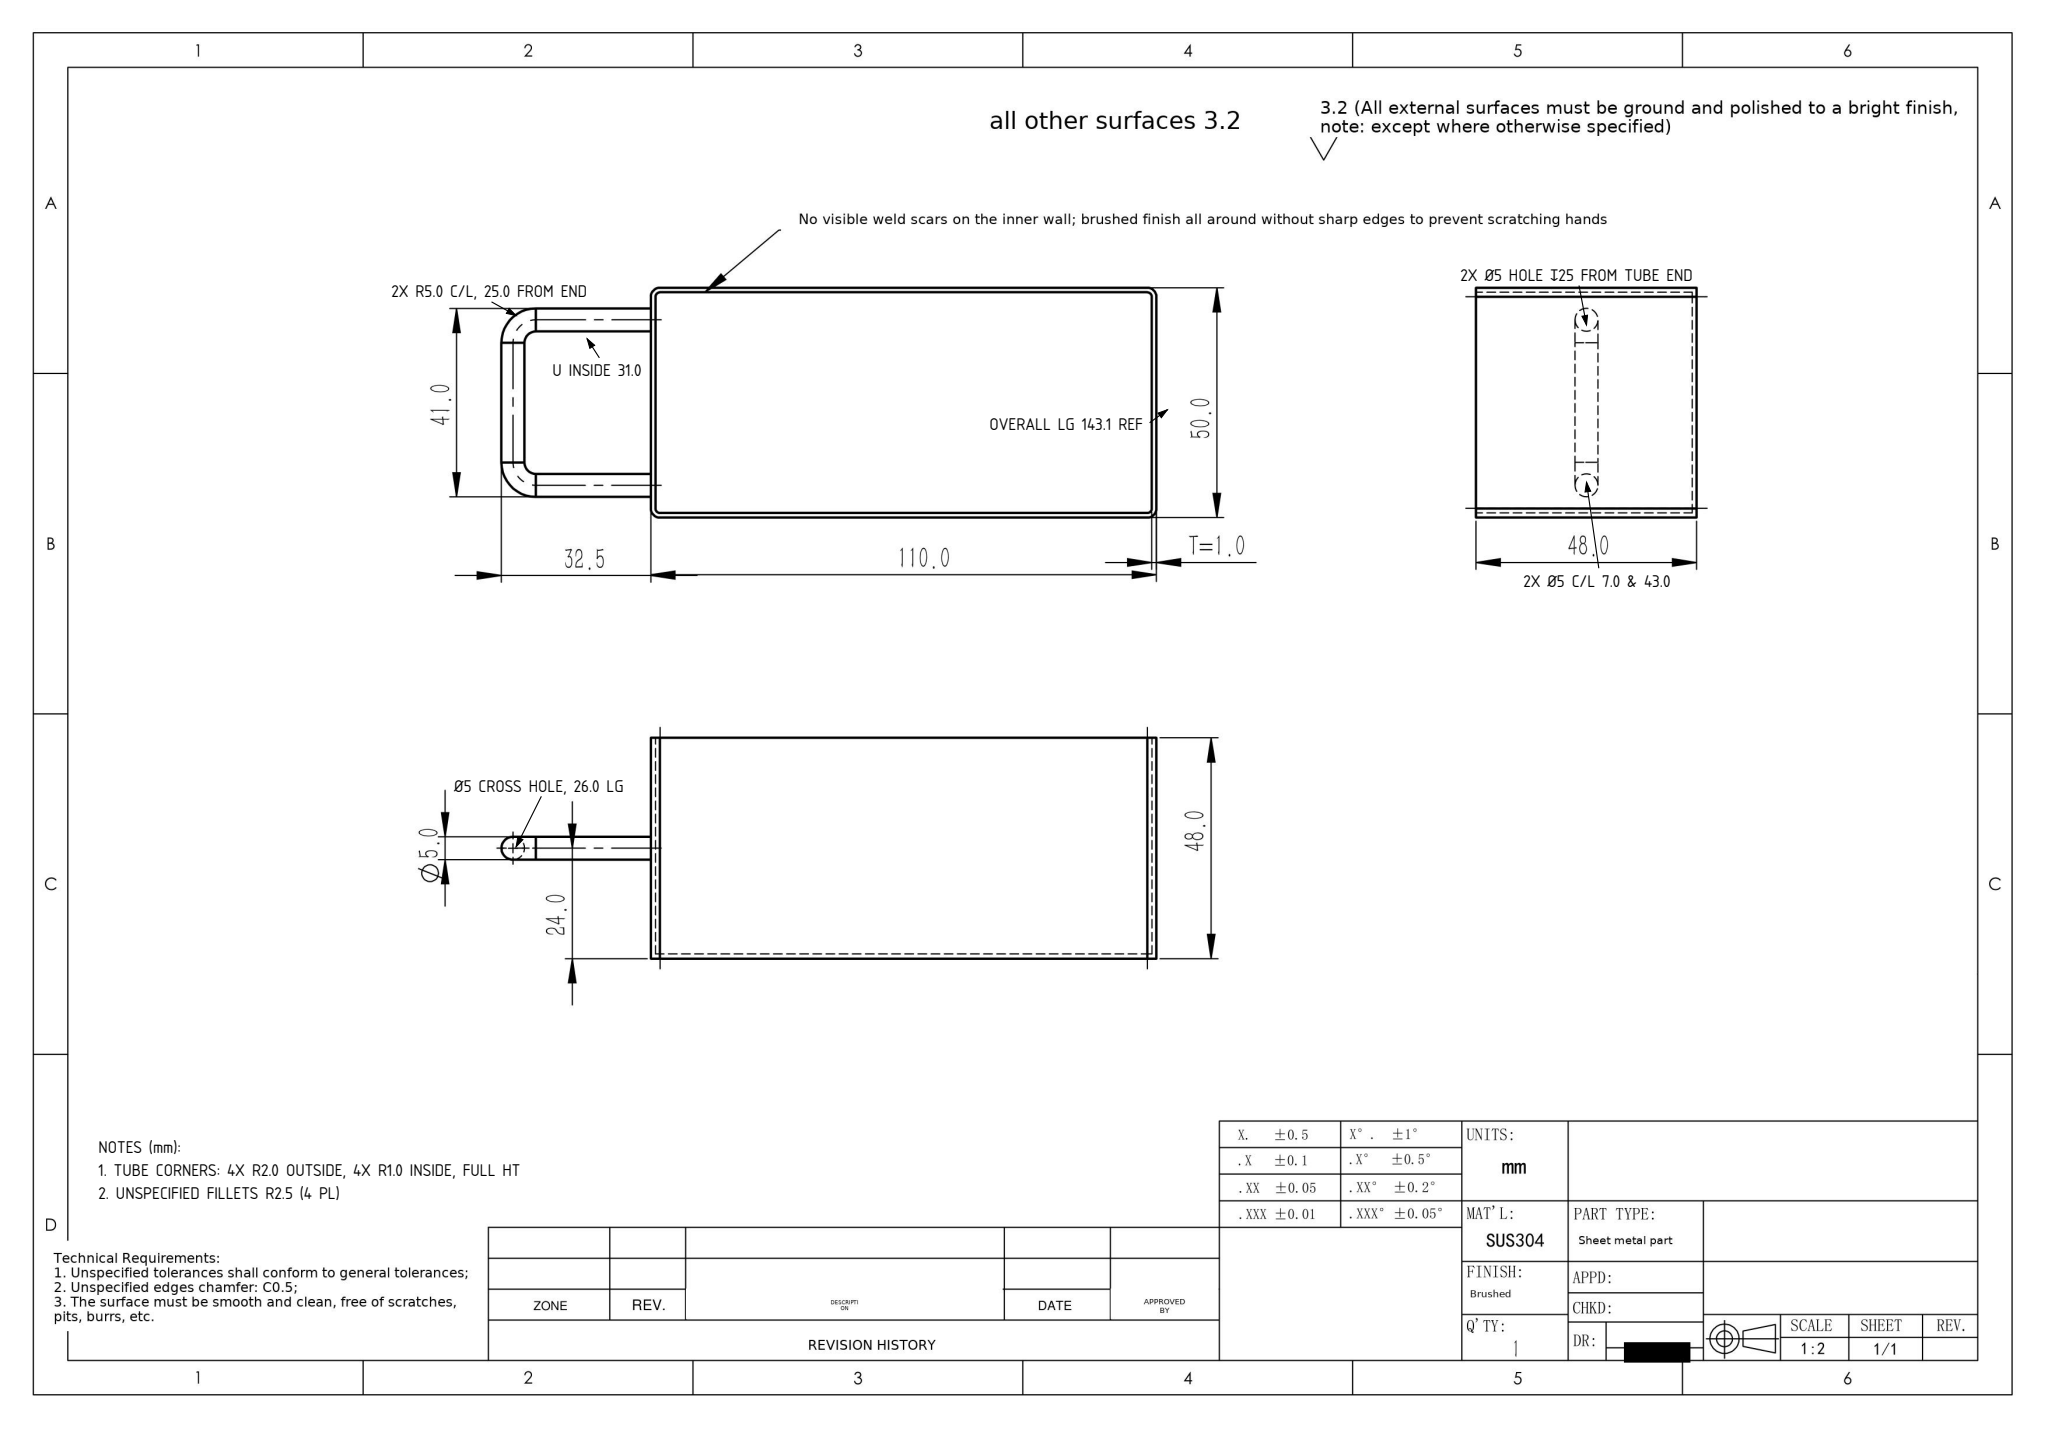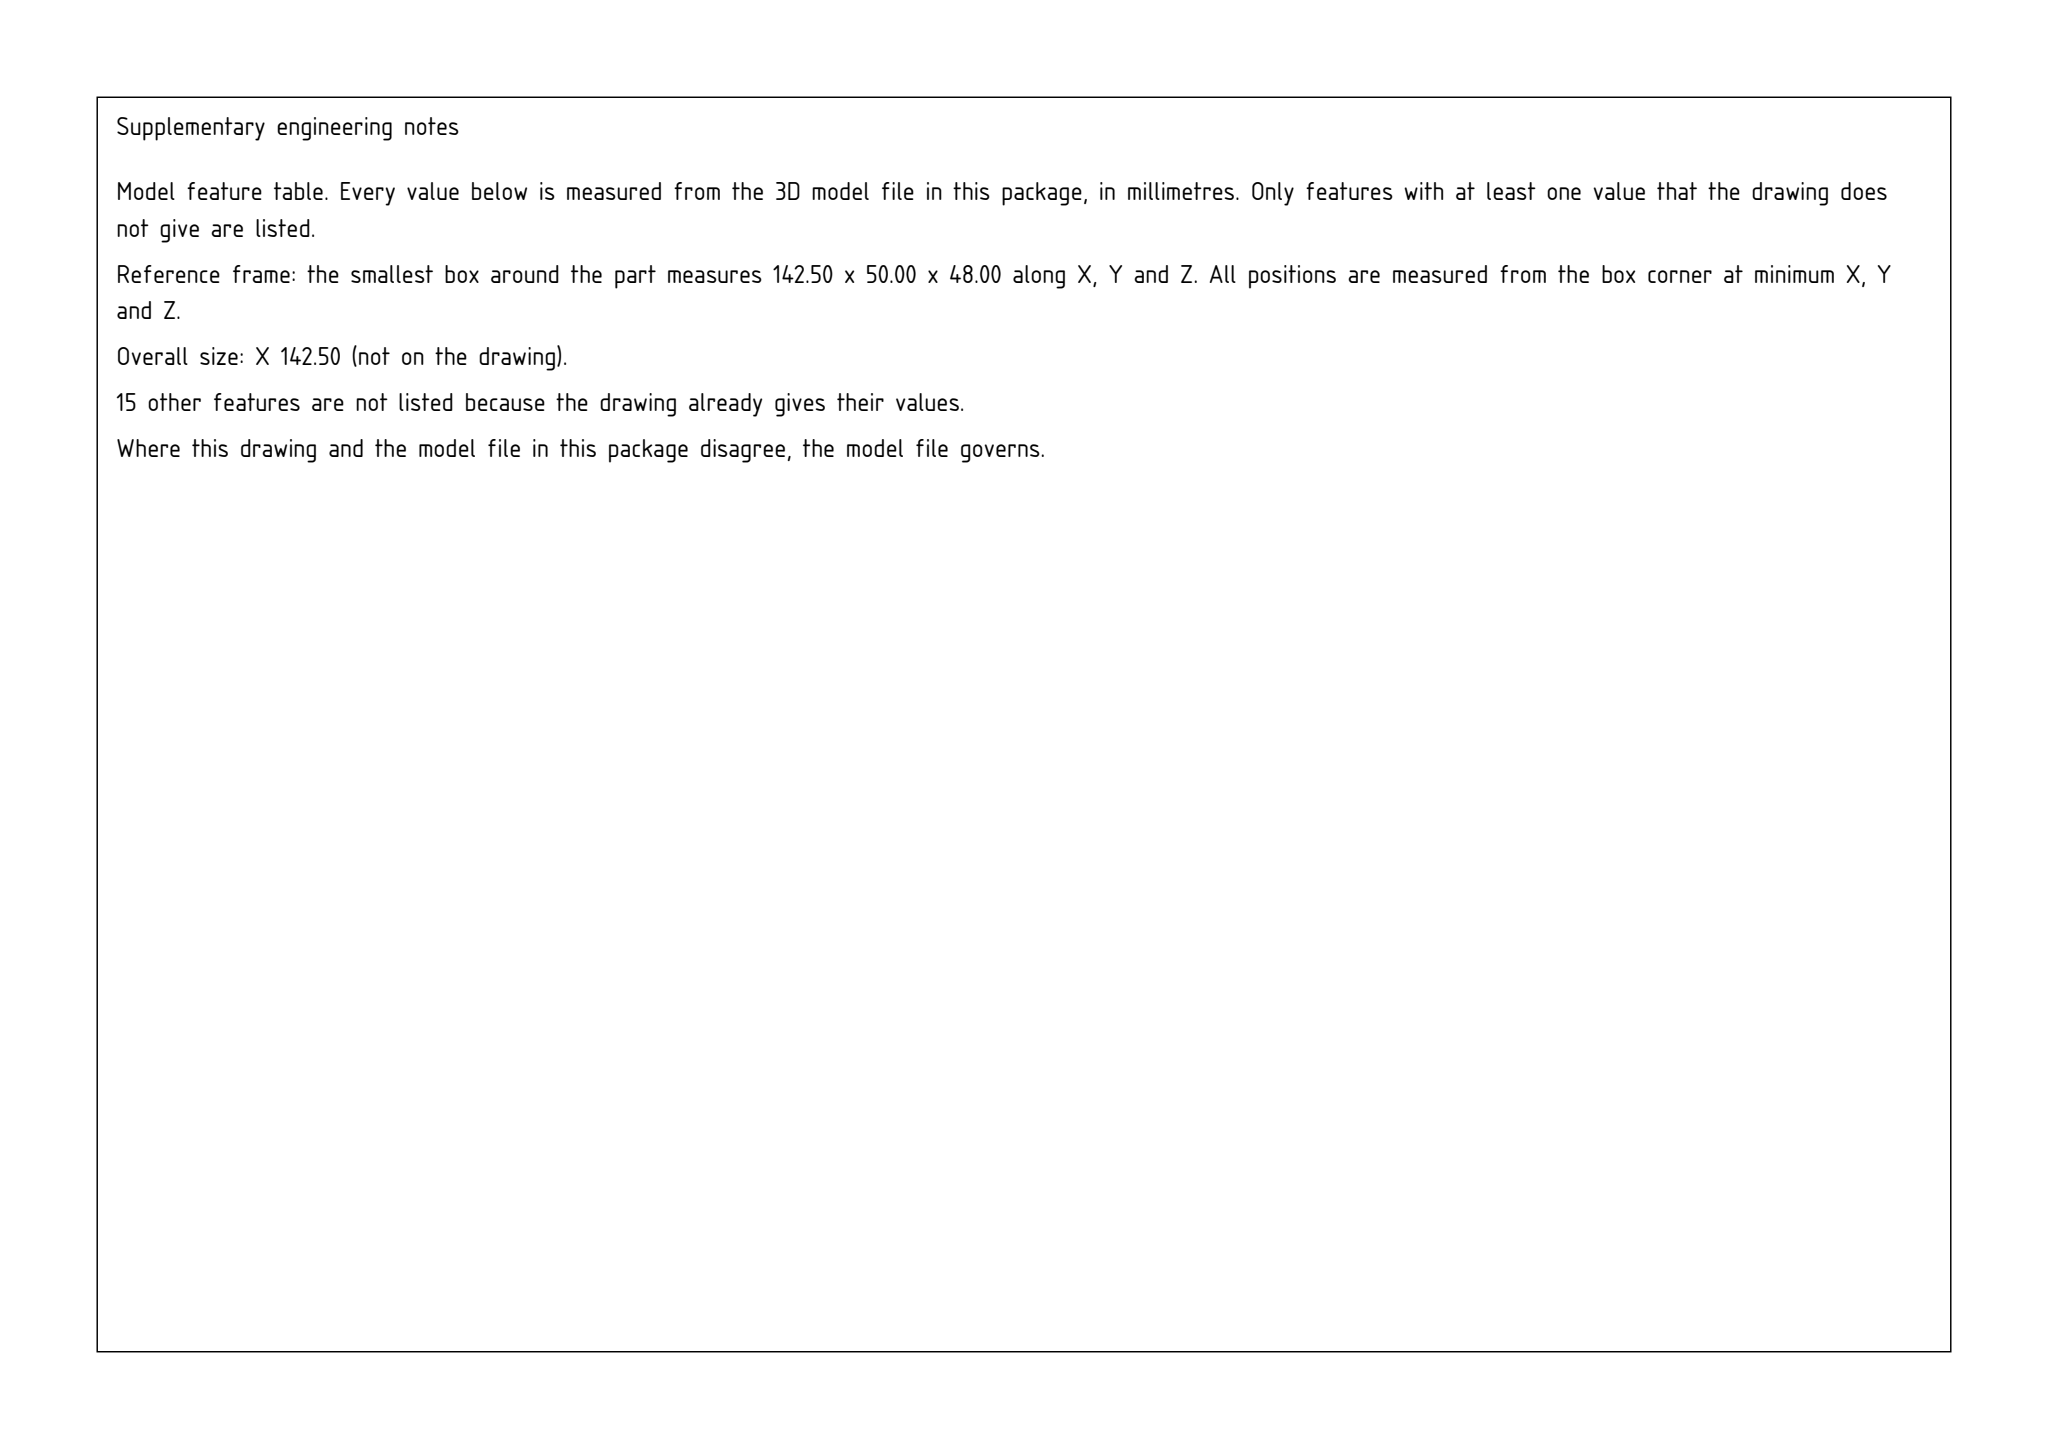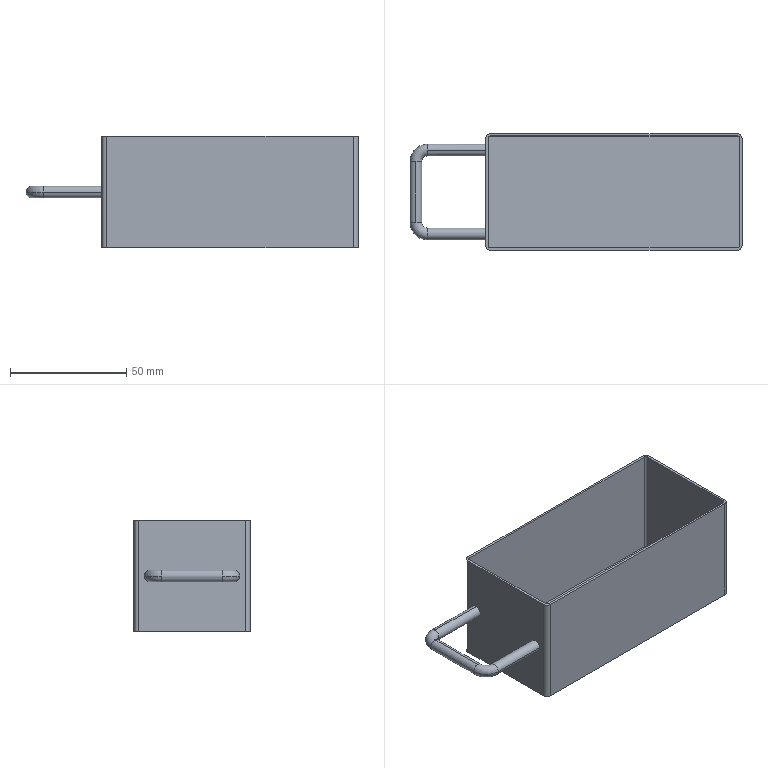Part | SolidWorks | mm | material SUS304 | 1 solid | 29 faces | box 142.5 x 50 x 48 mm | volume 22028 mm3 | cylinder 14 | plane 11 | torus 4 | commonest cylinder face diameters 5 x6 4 x4 2 x4
Drawing notes:
OVERALL LG 143.1 REF | from the solid: bbox_xyz X = 143.118 mm
2X Ø5 HOLE, 25.0 DP FROM 110.0 TUBE END FACE | from the solid: cyl dia 5.0 axis x, len 25.0, 2 ea; runs x=8.12 to tube face plane x=33.12
2X Ø5 HOLE C/L 7.0 & 43.0 FROM 50.0 SIDE FACES | from the solid: cyl dia 5.0 axis x at y=7.0 and y=43.0, z=24.0
Ø5 CROSS HOLE 26.0 LG, C/L 30.0 FROM TUBE END FACE | from the solid: cyl dia 5.0 axis y at x=3.12, z=24.0, len 26.0; 33.12-3.12=30.0
TUBE CORNERS: 4X R2.0 OUTSIDE, 4X R1.0 INSIDE, FULL HT | from the solid: dia 4.0 z-cyl len 48 and dia 2.0 z-cyl len 47 at (35.12/141.12, 2.0/48.0); tangent to faces x=33.12/143.12, y=0/50 and x=34.12/142.12, y=1/49
UNSPECIFIED FILLETS R2.5 (4 PL) | from the solid: fillet_radii [[2.5, 4]]
U-BEND R5.0 C/L, 2 PL; BEND C/L 25.0 FROM TUBE END FACE | from the solid: x-legs end x=8.12, cross hole axis x=3.12 (offset 5.0); cross len 26.0 = 36.0 c/c - 2x5.0
U INSIDE 31.0 (OUTSIDE 41.0 CTRD ON 50.0 WIDTH) | from the solid: leg c/l y=7.0 & 43.0, Ø5 tube: inside 36.0-5.0=31.0, outside 41.0, midpoint y=25.0